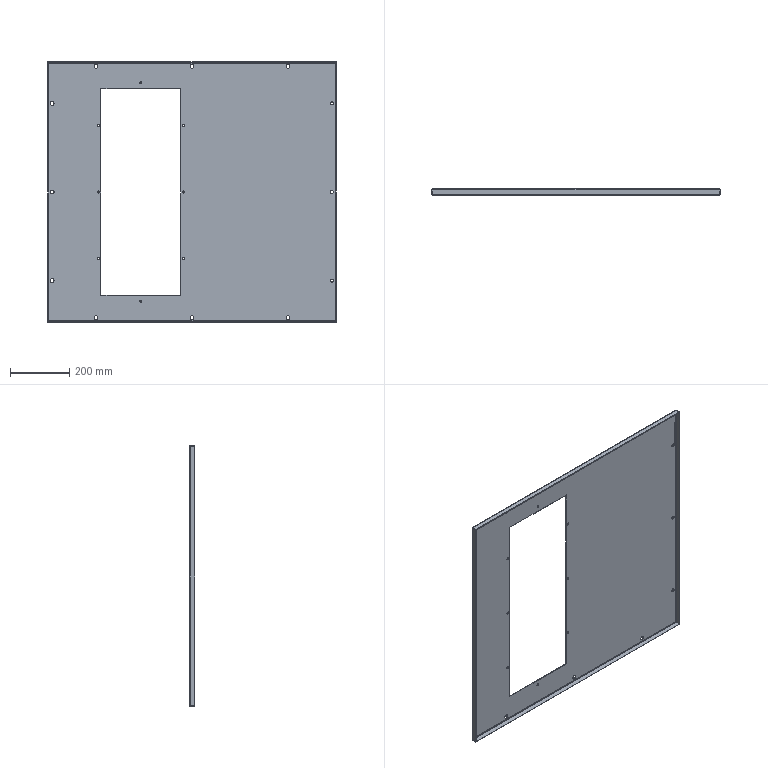Component | SolidWorks | Cover-1 | 1 solid | 90 faces | volume 1457326 mm3 | cylinder 48 | plane 34 | spline 8 | commonest cylinder face diameters 13 x18 7 x16 10 x6 4 x4 8 x4